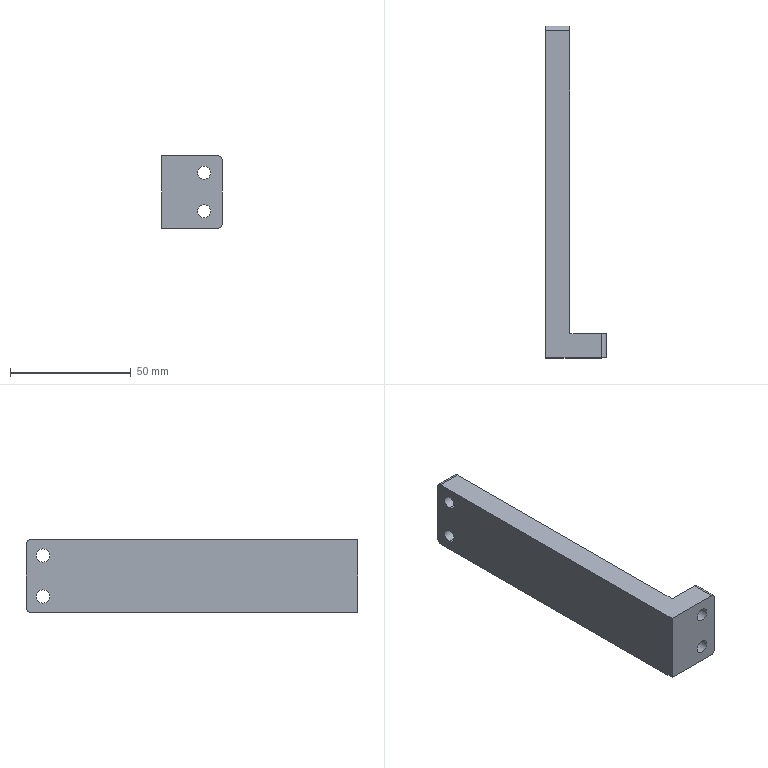Component | SolidWorks | ZHDJ-G002-1 | 1 solid | 32 faces | box 25 x 137.5 x 30 mm | volume 43516 mm3 | cylinder 20 | plane 12 | commonest cylinder face diameters 10 x8 5.5 x8 4 x4
build123d program:
from build123d import *

# Parameters (mm, degrees)
EXTRUDE_THIN1_DEPTH = 15
FILLET1_R           = 2


with BuildPart() as part:
    # Sketch1 → Extrude-Thin1 (new, symmetric)
    with BuildSketch(Plane(origin=(0, 0, 0), x_dir=(0, 0, -1), z_dir=(1, 0, 0))):
        Polygon((15, 0), (0, 0), (0, 127.5), (-10, 127.5), (-10, -10), (15, -10), align=None)
    extrude(amount=EXTRUDE_THIN1_DEPTH, both=True)

    # Fillet1
    fillet1_edges = [part.edges().sort_by_distance(p)[0] for p in [
        (15, 127.5, 5),
        (-15, 127.5, 5),
        (-15, -5, -15),
        (15, -5, -15),
    ]]
    fillet(fillet1_edges, radius=FILLET1_R)

    # Sketch3 → Hole Size _According to_ Type 1 of Hexag (revolve, cut)
    with BuildSketch(Plane(origin=(-8, 0, -7.5), x_dir=(0, 0, 1), z_dir=(1, 0, 0))):
        Polygon((0, 0), (0, 15.652), (2.75, 14), (2.75, 5.7), (5, 5.7), (5, 0), align=None)
    hole_size_according_to_type_1_of_hexag = revolve(axis=Axis((-8, 6.35, -7.5), (0, -1, 0)), mode=Mode.SUBTRACT)

    # Mirror1: Hole Size _According to_ Type 1 of Hexag across plane
    add(hole_size_according_to_type_1_of_hexag.mirror(Plane(origin=(0, 0, 0), x_dir=(0, 0, 1), z_dir=(1, 0, 0))), mode=Mode.SUBTRACT)

    # Sketch5 → Hole Size_ according to_ Type 2 Hex Sock (revolve, cut)
    with BuildSketch(Plane(origin=(8.5, 120.498, 0), x_dir=(0, 1, 0), z_dir=(1, 0, 0))):
        Polygon((0, 0), (0, 15.652), (2.75, 14), (2.75, 5.7), (5, 5.7), (5, 0), align=None)
    hole_size_according_to_type_2_hex_sock = revolve(axis=Axis((8.5, 120.498, -6.35), (0, 0, 1)), mode=Mode.SUBTRACT)

    # Mirror2: Hole Size_ according to_ Type 2 Hex Sock across plane
    add(hole_size_according_to_type_2_hex_sock.mirror(Plane(origin=(0, 0, 0), x_dir=(0, 0, 1), z_dir=(1, 0, 0))), mode=Mode.SUBTRACT)


solid = part.part

# Placed as in the assembly
solid = solid.moved(Location((56, -137.498, -110), (0, -90, 0)))
STEP:
#1=COLOUR_RGB('',0.7922,0.8196,0.9333);
#2=FILL_AREA_STYLE_COLOUR('',#1);
#3=FILL_AREA_STYLE('',(#2));
#4=SURFACE_STYLE_FILL_AREA(#3);
#5=SURFACE_SIDE_STYLE('',(#4));
#6=SURFACE_STYLE_USAGE(.BOTH.,#5);
#7=PRESENTATION_STYLE_ASSIGNMENT((#6));
#8=CARTESIAN_POINT('',(1.98,-0.6693,-4.469));
#9=VERTEX_POINT('',#8);
#10=CARTESIAN_POINT('',(1.98,-0.6693,-4.862));
#11=VERTEX_POINT('',#10);
#12=CARTESIAN_POINT('',(1.98,-0.6693,-4.665));
#13=DIRECTION('',(1.,0.,0.));
#14=DIRECTION('',(0.,0.,-1.));
#15=AXIS2_PLACEMENT_3D('',#12,#13,#14);
#16=CIRCLE('',#15,0.1969);
#17=EDGE_CURVE('',#9,#11,#16,.T.);
#18=ORIENTED_EDGE('',*,*,#17,.F.);
#19=CARTESIAN_POINT('',(2.205,-0.6693,-4.469));
#20=VERTEX_POINT('',#19);
#21=CARTESIAN_POINT('',(2.205,-0.6693,-4.469));
#22=DIRECTION('',(1.,0.,0.));
#23=VECTOR('',#22,39.37);
#24=LINE('',#21,#23);
#25=EDGE_CURVE('',#9,#20,#24,.T.);
#26=ORIENTED_EDGE('',*,*,#25,.T.);
#27=CARTESIAN_POINT('',(2.205,-0.6693,-4.862));
#28=VERTEX_POINT('',#27);
#29=CARTESIAN_POINT('',(2.205,-0.6693,-4.665));
#30=DIRECTION('',(1.,0.,0.));
#31=DIRECTION('',(0.,0.,-1.));
#32=AXIS2_PLACEMENT_3D('',#29,#30,#31);
#33=CIRCLE('',#32,0.1969);
#34=EDGE_CURVE('',#20,#28,#33,.T.);
#35=ORIENTED_EDGE('',*,*,#34,.T.);
#36=CARTESIAN_POINT('',(2.205,-0.6693,-4.862));
#37=DIRECTION('',(1.,0.,0.));
#38=VECTOR('',#37,39.37);
#39=LINE('',#36,#38);
#40=EDGE_CURVE('',#11,#28,#39,.T.);
#41=ORIENTED_EDGE('',*,*,#40,.F.);
#42=EDGE_LOOP('',(#18,#26,#35,#41));
#43=FACE_OUTER_BOUND('',#42,.T.);
#44=CARTESIAN_POINT('',(2.205,-0.6693,-4.665));
#45=DIRECTION('',(1.,0.,0.));
#46=DIRECTION('',(0.,0.,-1.));
#47=AXIS2_PLACEMENT_3D('',#44,#45,#46);
#48=CYLINDRICAL_SURFACE('',#47,0.1969);
#49=ADVANCED_FACE('',(#43),#48,.F.);
#50=CARTESIAN_POINT('',(1.811,-0.6693,-4.557));
#51=VERTEX_POINT('',#50);
#52=CARTESIAN_POINT('',(1.811,-0.6693,-4.774));
#53=VERTEX_POINT('',#52);
#54=CARTESIAN_POINT('',(1.811,-0.6693,-4.665));
#55=DIRECTION('',(1.,0.,0.));
#56=DIRECTION('',(0.,0.,-1.));
#57=AXIS2_PLACEMENT_3D('',#54,#55,#56);
#58=CIRCLE('',#57,0.1083);
#59=EDGE_CURVE('',#51,#53,#58,.T.);
#60=ORIENTED_EDGE('',*,*,#59,.F.);
#61=CARTESIAN_POINT('',(1.98,-0.6693,-4.557));
#62=VERTEX_POINT('',#61);
#63=CARTESIAN_POINT('',(2.205,-0.6693,-4.557));
#64=DIRECTION('',(1.,0.,0.));
#65=VECTOR('',#64,39.37);
#66=LINE('',#63,#65);
#67=EDGE_CURVE('',#51,#62,#66,.T.);
#68=ORIENTED_EDGE('',*,*,#67,.T.);
#69=CARTESIAN_POINT('',(1.98,-0.6693,-4.774));
#70=VERTEX_POINT('',#69);
#71=CARTESIAN_POINT('',(1.98,-0.6693,-4.665));
#72=DIRECTION('',(1.,0.,0.));
#73=DIRECTION('',(0.,0.,-1.));
#74=AXIS2_PLACEMENT_3D('',#71,#72,#73);
#75=CIRCLE('',#74,0.1083);
#76=EDGE_CURVE('',#62,#70,#75,.T.);
#77=ORIENTED_EDGE('',*,*,#76,.T.);
#78=CARTESIAN_POINT('',(2.205,-0.6693,-4.774));
#79=DIRECTION('',(1.,0.,0.));
#80=VECTOR('',#79,39.37);
#81=LINE('',#78,#80);
#82=EDGE_CURVE('',#53,#70,#81,.T.);
#83=ORIENTED_EDGE('',*,*,#82,.F.);
#84=EDGE_LOOP('',(#60,#68,#77,#83));
#85=FACE_OUTER_BOUND('',#84,.T.);
#86=CARTESIAN_POINT('',(2.205,-0.6693,-4.665));
#87=DIRECTION('',(1.,0.,0.));
#88=DIRECTION('',(0.,0.,-1.));
#89=AXIS2_PLACEMENT_3D('',#86,#87,#88);
#90=CYLINDRICAL_SURFACE('',#89,0.1083);
#91=ADVANCED_FACE('',(#85),#90,.F.);
#92=CARTESIAN_POINT('',(1.98,-0.6693,-3.799));
#93=VERTEX_POINT('',#92);
#94=CARTESIAN_POINT('',(1.98,-0.6693,-4.193));
#95=VERTEX_POINT('',#94);
#96=CARTESIAN_POINT('',(1.98,-0.6693,-3.996));
#97=DIRECTION('',(1.,0.,0.));
#98=DIRECTION('',(0.,0.,-1.));
#99=AXIS2_PLACEMENT_3D('',#96,#97,#98);
#100=CIRCLE('',#99,0.1969);
#101=EDGE_CURVE('',#93,#95,#100,.T.);
#102=ORIENTED_EDGE('',*,*,#101,.F.);
#103=CARTESIAN_POINT('',(2.205,-0.6693,-3.799));
#104=VERTEX_POINT('',#103);
#105=CARTESIAN_POINT('',(2.205,-0.6693,-3.799));
#106=DIRECTION('',(1.,0.,0.));
#107=VECTOR('',#106,39.37);
#108=LINE('',#105,#107);
#109=EDGE_CURVE('',#93,#104,#108,.T.);
#110=ORIENTED_EDGE('',*,*,#109,.T.);
#111=CARTESIAN_POINT('',(2.205,-0.6693,-4.193));
#112=VERTEX_POINT('',#111);
#113=CARTESIAN_POINT('',(2.205,-0.6693,-3.996));
#114=DIRECTION('',(1.,0.,0.));
#115=DIRECTION('',(0.,0.,-1.));
#116=AXIS2_PLACEMENT_3D('',#113,#114,#115);
#117=CIRCLE('',#116,0.1969);
#118=EDGE_CURVE('',#104,#112,#117,.T.);
#119=ORIENTED_EDGE('',*,*,#118,.T.);
#120=CARTESIAN_POINT('',(2.205,-0.6693,-4.193));
#121=DIRECTION('',(1.,0.,0.));
#122=VECTOR('',#121,39.37);
#123=LINE('',#120,#122);
#124=EDGE_CURVE('',#95,#112,#123,.T.);
#125=ORIENTED_EDGE('',*,*,#124,.F.);
#126=EDGE_LOOP('',(#102,#110,#119,#125));
#127=FACE_OUTER_BOUND('',#126,.T.);
#128=CARTESIAN_POINT('',(2.205,-0.6693,-3.996));
#129=DIRECTION('',(1.,0.,0.));
#130=DIRECTION('',(0.,0.,-1.));
#131=AXIS2_PLACEMENT_3D('',#128,#129,#130);
#132=CYLINDRICAL_SURFACE('',#131,0.1969);
#133=ADVANCED_FACE('',(#127),#132,.F.);
#134=CARTESIAN_POINT('',(1.811,-0.6693,-3.888));
#135=VERTEX_POINT('',#134);
#136=CARTESIAN_POINT('',(1.811,-0.6693,-4.104));
#137=VERTEX_POINT('',#136);
#138=CARTESIAN_POINT('',(1.811,-0.6693,-3.996));
#139=DIRECTION('',(1.,0.,0.));
#140=DIRECTION('',(0.,0.,-1.));
#141=AXIS2_PLACEMENT_3D('',#138,#139,#140);
#142=CIRCLE('',#141,0.1083);
#143=EDGE_CURVE('',#135,#137,#142,.T.);
#144=ORIENTED_EDGE('',*,*,#143,.F.);
#145=CARTESIAN_POINT('',(1.98,-0.6693,-3.888));
#146=VERTEX_POINT('',#145);
#147=CARTESIAN_POINT('',(2.205,-0.6693,-3.888));
#148=DIRECTION('',(1.,0.,0.));
#149=VECTOR('',#148,39.37);
#150=LINE('',#147,#149);
#151=EDGE_CURVE('',#135,#146,#150,.T.);
#152=ORIENTED_EDGE('',*,*,#151,.T.);
#153=CARTESIAN_POINT('',(1.98,-0.6693,-4.104));
#154=VERTEX_POINT('',#153);
#155=CARTESIAN_POINT('',(1.98,-0.6693,-3.996));
#156=DIRECTION('',(1.,0.,0.));
#157=DIRECTION('',(0.,0.,-1.));
#158=AXIS2_PLACEMENT_3D('',#155,#156,#157);
#159=CIRCLE('',#158,0.1083);
#160=EDGE_CURVE('',#146,#154,#159,.T.);
#161=ORIENTED_EDGE('',*,*,#160,.T.);
#162=CARTESIAN_POINT('',(2.205,-0.6693,-4.104));
#163=DIRECTION('',(1.,0.,0.));
#164=VECTOR('',#163,39.37);
#165=LINE('',#162,#164);
#166=EDGE_CURVE('',#137,#154,#165,.T.);
#167=ORIENTED_EDGE('',*,*,#166,.F.);
#168=EDGE_LOOP('',(#144,#152,#161,#167));
#169=FACE_OUTER_BOUND('',#168,.T.);
#170=CARTESIAN_POINT('',(2.205,-0.6693,-3.996));
#171=DIRECTION('',(1.,0.,0.));
#172=DIRECTION('',(0.,0.,-1.));
#173=AXIS2_PLACEMENT_3D('',#170,#171,#172);
#174=CYLINDRICAL_SURFACE('',#173,0.1083);
#175=ADVANCED_FACE('',(#169),#174,.F.);
#176=CARTESIAN_POINT('',(2.697,-5.638,-4.016));
#177=VERTEX_POINT('',#176);
#178=CARTESIAN_POINT('',(2.303,-5.638,-4.016));
#179=VERTEX_POINT('',#178);
#180=CARTESIAN_POINT('',(2.5,-5.638,-4.016));
#181=DIRECTION('',(0.,1.,0.));
#182=DIRECTION('',(-1.,0.,0.));
#183=AXIS2_PLACEMENT_3D('',#180,#181,#182);
#184=CIRCLE('',#183,0.1969);
#185=EDGE_CURVE('',#177,#179,#184,.T.);
#186=ORIENTED_EDGE('',*,*,#185,.F.);
#187=CARTESIAN_POINT('',(2.697,-5.413,-4.016));
#188=VERTEX_POINT('',#187);
#189=CARTESIAN_POINT('',(2.697,-5.413,-4.016));
#190=DIRECTION('',(0.,1.,0.));
#191=VECTOR('',#190,39.37);
#192=LINE('',#189,#191);
#193=EDGE_CURVE('',#177,#188,#192,.T.);
#194=ORIENTED_EDGE('',*,*,#193,.T.);
#195=CARTESIAN_POINT('',(2.303,-5.413,-4.016));
#196=VERTEX_POINT('',#195);
#197=CARTESIAN_POINT('',(2.5,-5.413,-4.016));
#198=DIRECTION('',(0.,1.,0.));
#199=DIRECTION('',(-1.,0.,0.));
#200=AXIS2_PLACEMENT_3D('',#197,#198,#199);
#201=CIRCLE('',#200,0.1969);
#202=EDGE_CURVE('',#188,#196,#201,.T.);
#203=ORIENTED_EDGE('',*,*,#202,.T.);
#204=CARTESIAN_POINT('',(2.303,-5.413,-4.016));
#205=DIRECTION('',(0.,1.,0.));
#206=VECTOR('',#205,39.37);
#207=LINE('',#204,#206);
#208=EDGE_CURVE('',#179,#196,#207,.T.);
#209=ORIENTED_EDGE('',*,*,#208,.F.);
#210=EDGE_LOOP('',(#186,#194,#203,#209));
#211=FACE_OUTER_BOUND('',#210,.T.);
#212=CARTESIAN_POINT('',(2.5,-5.413,-4.016));
#213=DIRECTION('',(0.,1.,0.));
#214=DIRECTION('',(-1.,0.,0.));
#215=AXIS2_PLACEMENT_3D('',#212,#213,#214);
#216=CYLINDRICAL_SURFACE('',#215,0.1969);
#217=ADVANCED_FACE('',(#211),#216,.F.);
#218=CARTESIAN_POINT('',(2.608,-5.807,-4.016));
#219=VERTEX_POINT('',#218);
#220=CARTESIAN_POINT('',(2.392,-5.807,-4.016));
#221=VERTEX_POINT('',#220);
#222=CARTESIAN_POINT('',(2.5,-5.807,-4.016));
#223=DIRECTION('',(0.,1.,0.));
#224=DIRECTION('',(-1.,0.,0.));
#225=AXIS2_PLACEMENT_3D('',#222,#223,#224);
#226=CIRCLE('',#225,0.1083);
#227=EDGE_CURVE('',#219,#221,#226,.T.);
#228=ORIENTED_EDGE('',*,*,#227,.F.);
#229=CARTESIAN_POINT('',(2.608,-5.638,-4.016));
#230=VERTEX_POINT('',#229);
#231=CARTESIAN_POINT('',(2.608,-5.413,-4.016));
#232=DIRECTION('',(0.,1.,0.));
#233=VECTOR('',#232,39.37);
#234=LINE('',#231,#233);
#235=EDGE_CURVE('',#219,#230,#234,.T.);
#236=ORIENTED_EDGE('',*,*,#235,.T.);
#237=CARTESIAN_POINT('',(2.392,-5.638,-4.016));
#238=VERTEX_POINT('',#237);
#239=CARTESIAN_POINT('',(2.5,-5.638,-4.016));
#240=DIRECTION('',(0.,1.,0.));
#241=DIRECTION('',(-1.,0.,0.));
#242=AXIS2_PLACEMENT_3D('',#239,#240,#241);
#243=CIRCLE('',#242,0.1083);
#244=EDGE_CURVE('',#230,#238,#243,.T.);
#245=ORIENTED_EDGE('',*,*,#244,.T.);
#246=CARTESIAN_POINT('',(2.392,-5.413,-4.016));
#247=DIRECTION('',(0.,1.,0.));
#248=VECTOR('',#247,39.37);
#249=LINE('',#246,#248);
#250=EDGE_CURVE('',#221,#238,#249,.T.);
#251=ORIENTED_EDGE('',*,*,#250,.F.);
#252=EDGE_LOOP('',(#228,#236,#245,#251));
#253=FACE_OUTER_BOUND('',#252,.T.);
#254=CARTESIAN_POINT('',(2.5,-5.413,-4.016));
#255=DIRECTION('',(0.,1.,0.));
#256=DIRECTION('',(-1.,0.,0.));
#257=AXIS2_PLACEMENT_3D('',#254,#255,#256);
#258=CYLINDRICAL_SURFACE('',#257,0.1083);
#259=ADVANCED_FACE('',(#253),#258,.F.);
#260=CARTESIAN_POINT('',(2.697,-5.638,-4.646));
#261=VERTEX_POINT('',#260);
#262=CARTESIAN_POINT('',(2.303,-5.638,-4.646));
#263=VERTEX_POINT('',#262);
#264=CARTESIAN_POINT('',(2.5,-5.638,-4.646));
#265=DIRECTION('',(0.,1.,0.));
#266=DIRECTION('',(-1.,0.,0.));
#267=AXIS2_PLACEMENT_3D('',#264,#265,#266);
#268=CIRCLE('',#267,0.1969);
#269=EDGE_CURVE('',#261,#263,#268,.T.);
#270=ORIENTED_EDGE('',*,*,#269,.F.);
#271=CARTESIAN_POINT('',(2.697,-5.413,-4.646));
#272=VERTEX_POINT('',#271);
#273=CARTESIAN_POINT('',(2.697,-5.413,-4.646));
#274=DIRECTION('',(0.,1.,0.));
#275=VECTOR('',#274,39.37);
#276=LINE('',#273,#275);
#277=EDGE_CURVE('',#261,#272,#276,.T.);
#278=ORIENTED_EDGE('',*,*,#277,.T.);
#279=CARTESIAN_POINT('',(2.303,-5.413,-4.646));
#280=VERTEX_POINT('',#279);
#281=CARTESIAN_POINT('',(2.5,-5.413,-4.646));
#282=DIRECTION('',(0.,1.,0.));
#283=DIRECTION('',(-1.,0.,0.));
#284=AXIS2_PLACEMENT_3D('',#281,#282,#283);
#285=CIRCLE('',#284,0.1969);
#286=EDGE_CURVE('',#272,#280,#285,.T.);
#287=ORIENTED_EDGE('',*,*,#286,.T.);
#288=CARTESIAN_POINT('',(2.303,-5.413,-4.646));
#289=DIRECTION('',(0.,1.,0.));
#290=VECTOR('',#289,39.37);
#291=LINE('',#288,#290);
#292=EDGE_CURVE('',#263,#280,#291,.T.);
#293=ORIENTED_EDGE('',*,*,#292,.F.);
#294=EDGE_LOOP('',(#270,#278,#287,#293));
#295=FACE_OUTER_BOUND('',#294,.T.);
#296=CARTESIAN_POINT('',(2.5,-5.413,-4.646));
#297=DIRECTION('',(0.,1.,0.));
#298=DIRECTION('',(-1.,0.,0.));
#299=AXIS2_PLACEMENT_3D('',#296,#297,#298);
#300=CYLINDRICAL_SURFACE('',#299,0.1969);
#301=ADVANCED_FACE('',(#295),#300,.F.);
#302=CARTESIAN_POINT('',(2.608,-5.807,-4.646));
#303=VERTEX_POINT('',#302);
#304=CARTESIAN_POINT('',(2.392,-5.807,-4.646));
#305=VERTEX_POINT('',#304);
#306=CARTESIAN_POINT('',(2.5,-5.807,-4.646));
#307=DIRECTION('',(0.,1.,0.));
#308=DIRECTION('',(-1.,0.,0.));
#309=AXIS2_PLACEMENT_3D('',#306,#307,#308);
#310=CIRCLE('',#309,0.1083);
#311=EDGE_CURVE('',#303,#305,#310,.T.);
#312=ORIENTED_EDGE('',*,*,#311,.F.);
#313=CARTESIAN_POINT('',(2.608,-5.638,-4.646));
#314=VERTEX_POINT('',#313);
#315=CARTESIAN_POINT('',(2.608,-5.413,-4.646));
#316=DIRECTION('',(0.,1.,0.));
#317=VECTOR('',#316,39.37);
#318=LINE('',#315,#317);
#319=EDGE_CURVE('',#303,#314,#318,.T.);
#320=ORIENTED_EDGE('',*,*,#319,.T.);
#321=CARTESIAN_POINT('',(2.392,-5.638,-4.646));
#322=VERTEX_POINT('',#321);
#323=CARTESIAN_POINT('',(2.5,-5.638,-4.646));
#324=DIRECTION('',(0.,1.,0.));
#325=DIRECTION('',(-1.,0.,0.));
#326=AXIS2_PLACEMENT_3D('',#323,#324,#325);
#327=CIRCLE('',#326,0.1083);
#328=EDGE_CURVE('',#314,#322,#327,.T.);
#329=ORIENTED_EDGE('',*,*,#328,.T.);
#330=CARTESIAN_POINT('',(2.392,-5.413,-4.646));
#331=DIRECTION('',(0.,1.,0.));
#332=VECTOR('',#331,39.37);
#333=LINE('',#330,#332);
#334=EDGE_CURVE('',#305,#322,#333,.T.);
#335=ORIENTED_EDGE('',*,*,#334,.F.);
#336=EDGE_LOOP('',(#312,#320,#329,#335));
#337=FACE_OUTER_BOUND('',#336,.T.);
#338=CARTESIAN_POINT('',(2.5,-5.413,-4.646));
#339=DIRECTION('',(0.,1.,0.));
#340=DIRECTION('',(-1.,0.,0.));
#341=AXIS2_PLACEMENT_3D('',#338,#339,#340);
#342=CYLINDRICAL_SURFACE('',#341,0.1083);
#343=ADVANCED_FACE('',(#337),#342,.F.);
#344=CARTESIAN_POINT('',(2.5,-5.807,-4.016));
#345=DIRECTION('',(0.,1.,0.));
#346=DIRECTION('',(-1.,0.,0.));
#347=AXIS2_PLACEMENT_3D('',#344,#345,#346);
#348=CIRCLE('',#347,0.1083);
#349=EDGE_CURVE('',#221,#219,#348,.T.);
#350=ORIENTED_EDGE('',*,*,#349,.T.);
#351=ORIENTED_EDGE('',*,*,#227,.T.);
#352=EDGE_LOOP('',(#350,#351));
#353=FACE_BOUND('',#352,.T.);
#354=CARTESIAN_POINT('',(2.5,-5.807,-4.646));
#355=DIRECTION('',(0.,1.,0.));
#356=DIRECTION('',(-1.,0.,0.));
#357=AXIS2_PLACEMENT_3D('',#354,#355,#356);
#358=CIRCLE('',#357,0.1083);
#359=EDGE_CURVE('',#305,#303,#358,.T.);
#360=ORIENTED_EDGE('',*,*,#359,.T.);
#361=ORIENTED_EDGE('',*,*,#311,.T.);
#362=EDGE_LOOP('',(#360,#361));
#363=FACE_BOUND('',#362,.T.);
#364=CARTESIAN_POINT('',(2.795,-5.807,-3.819));
#365=VERTEX_POINT('',#364);
#366=CARTESIAN_POINT('',(2.795,-5.807,-4.843));
#367=VERTEX_POINT('',#366);
#368=CARTESIAN_POINT('',(2.795,-5.807,-3.74));
#369=DIRECTION('',(0.,0.,-1.));
#370=VECTOR('',#369,39.37);
#371=LINE('',#368,#370);
#372=EDGE_CURVE('',#365,#367,#371,.T.);
#373=ORIENTED_EDGE('',*,*,#372,.F.);
#374=CARTESIAN_POINT('',(2.717,-5.807,-3.74));
#375=VERTEX_POINT('',#374);
#376=CARTESIAN_POINT('',(2.717,-5.807,-3.819));
#377=DIRECTION('',(0.,-1.,0.));
#378=DIRECTION('',(-1.,0.,0.));
#379=AXIS2_PLACEMENT_3D('',#376,#377,#378);
#380=CIRCLE('',#379,0.07874);
#381=EDGE_CURVE('',#365,#375,#380,.T.);
#382=ORIENTED_EDGE('',*,*,#381,.T.);
#383=CARTESIAN_POINT('',(1.811,-5.807,-3.74));
#384=VERTEX_POINT('',#383);
#385=CARTESIAN_POINT('',(2.205,-5.807,-3.74));
#386=DIRECTION('',(1.,0.,0.));
#387=VECTOR('',#386,39.37);
#388=LINE('',#385,#387);
#389=EDGE_CURVE('',#384,#375,#388,.T.);
#390=ORIENTED_EDGE('',*,*,#389,.F.);
#391=CARTESIAN_POINT('',(1.811,-5.807,-4.921));
#392=VERTEX_POINT('',#391);
#393=CARTESIAN_POINT('',(1.811,-5.807,-3.74));
#394=DIRECTION('',(0.,0.,-1.));
#395=VECTOR('',#394,39.37);
#396=LINE('',#393,#395);
#397=EDGE_CURVE('',#384,#392,#396,.T.);
#398=ORIENTED_EDGE('',*,*,#397,.T.);
#399=CARTESIAN_POINT('',(2.717,-5.807,-4.921));
#400=VERTEX_POINT('',#399);
#401=CARTESIAN_POINT('',(2.205,-5.807,-4.921));
#402=DIRECTION('',(1.,0.,0.));
#403=VECTOR('',#402,39.37);
#404=LINE('',#401,#403);
#405=EDGE_CURVE('',#392,#400,#404,.T.);
#406=ORIENTED_EDGE('',*,*,#405,.T.);
#407=CARTESIAN_POINT('',(2.717,-5.807,-4.843));
#408=DIRECTION('',(0.,-1.,0.));
#409=DIRECTION('',(-1.,0.,0.));
#410=AXIS2_PLACEMENT_3D('',#407,#408,#409);
#411=CIRCLE('',#410,0.07874);
#412=EDGE_CURVE('',#400,#367,#411,.T.);
#413=ORIENTED_EDGE('',*,*,#412,.T.);
#414=EDGE_LOOP('',(#373,#382,#390,#398,#406,#413));
#415=FACE_OUTER_BOUND('',#414,.T.);
#416=CARTESIAN_POINT('',(2.205,-5.807,-3.74));
#417=DIRECTION('',(0.,1.,0.));
#418=DIRECTION('',(-1.,0.,0.));
#419=AXIS2_PLACEMENT_3D('',#416,#417,#418);
#420=PLANE('',#419);
#421=ADVANCED_FACE('',(#353,#363,#415),#420,.F.);
#422=CARTESIAN_POINT('',(2.795,-5.413,-3.819));
#423=VERTEX_POINT('',#422);
#424=CARTESIAN_POINT('',(2.795,-5.413,-4.843));
#425=VERTEX_POINT('',#424);
#426=CARTESIAN_POINT('',(2.795,-5.413,-3.74));
#427=DIRECTION('',(0.,0.,-1.));
#428=VECTOR('',#427,39.37);
#429=LINE('',#426,#428);
#430=EDGE_CURVE('',#423,#425,#429,.T.);
#431=ORIENTED_EDGE('',*,*,#430,.F.);
#432=CARTESIAN_POINT('',(2.795,-5.807,-3.819));
#433=DIRECTION('',(0.,-1.,0.));
#434=VECTOR('',#433,39.37);
#435=LINE('',#432,#434);
#436=EDGE_CURVE('',#423,#365,#435,.T.);
#437=ORIENTED_EDGE('',*,*,#436,.T.);
#438=ORIENTED_EDGE('',*,*,#372,.T.);
#439=CARTESIAN_POINT('',(2.795,-5.413,-4.843));
#440=DIRECTION('',(0.,1.,0.));
#441=VECTOR('',#440,39.37);
#442=LINE('',#439,#441);
#443=EDGE_CURVE('',#367,#425,#442,.T.);
#444=ORIENTED_EDGE('',*,*,#443,.T.);
#445=EDGE_LOOP('',(#431,#437,#438,#444));
#446=FACE_OUTER_BOUND('',#445,.T.);
#447=CARTESIAN_POINT('',(2.795,-5.413,-3.74));
#448=DIRECTION('',(1.,0.,0.));
#449=DIRECTION('',(0.,0.,-1.));
#450=AXIS2_PLACEMENT_3D('',#447,#448,#449);
#451=PLANE('',#450);
#452=ADVANCED_FACE('',(#446),#451,.T.);
#453=CARTESIAN_POINT('',(2.5,-5.413,-4.016));
#454=DIRECTION('',(0.,1.,0.));
#455=DIRECTION('',(-1.,0.,0.));
#456=AXIS2_PLACEMENT_3D('',#453,#454,#455);
#457=CIRCLE('',#456,0.1969);
#458=EDGE_CURVE('',#196,#188,#457,.T.);
#459=ORIENTED_EDGE('',*,*,#458,.F.);
#460=ORIENTED_EDGE('',*,*,#202,.F.);
#461=EDGE_LOOP('',(#459,#460));
#462=FACE_BOUND('',#461,.T.);
#463=CARTESIAN_POINT('',(2.5,-5.413,-4.646));
#464=DIRECTION('',(0.,1.,0.));
#465=DIRECTION('',(-1.,0.,0.));
#466=AXIS2_PLACEMENT_3D('',#463,#464,#465);
#467=CIRCLE('',#466,0.1969);
#468=EDGE_CURVE('',#280,#272,#467,.T.);
#469=ORIENTED_EDGE('',*,*,#468,.F.);
#470=ORIENTED_EDGE('',*,*,#286,.F.);
#471=EDGE_LOOP('',(#469,#470));
#472=FACE_BOUND('',#471,.T.);
#473=CARTESIAN_POINT('',(2.205,-5.413,-3.74));
#474=VERTEX_POINT('',#473);
#475=CARTESIAN_POINT('',(2.717,-5.413,-3.74));
#476=VERTEX_POINT('',#475);
#477=CARTESIAN_POINT('',(2.205,-5.413,-3.74));
#478=DIRECTION('',(1.,0.,0.));
#479=VECTOR('',#478,39.37);
#480=LINE('',#477,#479);
#481=EDGE_CURVE('',#474,#476,#480,.T.);
#482=ORIENTED_EDGE('',*,*,#481,.T.);
#483=CARTESIAN_POINT('',(2.717,-5.413,-3.819));
#484=DIRECTION('',(0.,1.,0.));
#485=DIRECTION('',(-1.,0.,0.));
#486=AXIS2_PLACEMENT_3D('',#483,#484,#485);
#487=CIRCLE('',#486,0.07874);
#488=EDGE_CURVE('',#476,#423,#487,.T.);
#489=ORIENTED_EDGE('',*,*,#488,.T.);
#490=ORIENTED_EDGE('',*,*,#430,.T.);
#491=CARTESIAN_POINT('',(2.717,-5.413,-4.921));
#492=VERTEX_POINT('',#491);
#493=CARTESIAN_POINT('',(2.717,-5.413,-4.843));
#494=DIRECTION('',(0.,1.,0.));
#495=DIRECTION('',(-1.,0.,0.));
#496=AXIS2_PLACEMENT_3D('',#493,#494,#495);
#497=CIRCLE('',#496,0.07874);
#498=EDGE_CURVE('',#425,#492,#497,.T.);
#499=ORIENTED_EDGE('',*,*,#498,.T.);
#500=CARTESIAN_POINT('',(2.205,-5.413,-4.921));
#501=VERTEX_POINT('',#500);
#502=CARTESIAN_POINT('',(2.205,-5.413,-4.921));
#503=DIRECTION('',(1.,0.,0.));
#504=VECTOR('',#503,39.37);
#505=LINE('',#502,#504);
#506=EDGE_CURVE('',#501,#492,#505,.T.);
#507=ORIENTED_EDGE('',*,*,#506,.F.);
#508=CARTESIAN_POINT('',(2.205,-5.413,-3.74));
#509=DIRECTION('',(0.,0.,-1.));
#510=VECTOR('',#509,39.37);
#511=LINE('',#508,#510);
#512=EDGE_CURVE('',#474,#501,#511,.T.);
#513=ORIENTED_EDGE('',*,*,#512,.F.);
#514=EDGE_LOOP('',(#482,#489,#490,#499,#507,#513));
#515=FACE_OUTER_BOUND('',#514,.T.);
#516=CARTESIAN_POINT('',(2.205,-5.413,-3.74));
#517=DIRECTION('',(0.,1.,0.));
#518=DIRECTION('',(-1.,0.,0.));
#519=AXIS2_PLACEMENT_3D('',#516,#517,#518);
#520=PLANE('',#519);
#521=ADVANCED_FACE('',(#462,#472,#515),#520,.T.);
#522=CARTESIAN_POINT('',(2.205,-0.6693,-4.665));
#523=DIRECTION('',(1.,0.,0.));
#524=DIRECTION('',(0.,0.,-1.));
#525=AXIS2_PLACEMENT_3D('',#522,#523,#524);
#526=CIRCLE('',#525,0.1969);
#527=EDGE_CURVE('',#28,#20,#526,.T.);
#528=ORIENTED_EDGE('',*,*,#527,.F.);
#529=ORIENTED_EDGE('',*,*,#34,.F.);
#530=EDGE_LOOP('',(#528,#529));
#531=FACE_BOUND('',#530,.T.);
#532=CARTESIAN_POINT('',(2.205,-0.6693,-3.996));
#533=DIRECTION('',(1.,0.,0.));
#534=DIRECTION('',(0.,0.,-1.));
#535=AXIS2_PLACEMENT_3D('',#532,#533,#534);
#536=CIRCLE('',#535,0.1969);
#537=EDGE_CURVE('',#112,#104,#536,.T.);
#538=ORIENTED_EDGE('',*,*,#537,.F.);
#539=ORIENTED_EDGE('',*,*,#118,.F.);
#540=EDGE_LOOP('',(#538,#539));
#541=FACE_BOUND('',#540,.T.);
#542=CARTESIAN_POINT('',(2.205,-0.4724,-4.921));
#543=VERTEX_POINT('',#542);
#544=CARTESIAN_POINT('',(2.205,-5.413,-4.921));
#545=DIRECTION('',(0.,-1.,0.));
#546=VECTOR('',#545,39.37);
#547=LINE('',#544,#546);
#548=EDGE_CURVE('',#543,#501,#547,.T.);
#549=ORIENTED_EDGE('',*,*,#548,.F.);
#550=CARTESIAN_POINT('',(2.205,-0.3936,-4.843));
#551=VERTEX_POINT('',#550);
#552=CARTESIAN_POINT('',(2.205,-0.4724,-4.843));
#553=DIRECTION('',(1.,0.,0.));
#554=DIRECTION('',(0.,0.,-1.));
#555=AXIS2_PLACEMENT_3D('',#552,#553,#554);
#556=CIRCLE('',#555,0.07874);
#557=EDGE_CURVE('',#543,#551,#556,.T.);
#558=ORIENTED_EDGE('',*,*,#557,.T.);
#559=CARTESIAN_POINT('',(2.205,-0.3936,-3.819));
#560=VERTEX_POINT('',#559);
#561=CARTESIAN_POINT('',(2.205,-0.3936,-3.74));
#562=DIRECTION('',(0.,0.,-1.));
#563=VECTOR('',#562,39.37);
#564=LINE('',#561,#563);
#565=EDGE_CURVE('',#560,#551,#564,.T.);
#566=ORIENTED_EDGE('',*,*,#565,.F.);
#567=CARTESIAN_POINT('',(2.205,-0.4724,-3.74));
#568=VERTEX_POINT('',#567);
#569=CARTESIAN_POINT('',(2.205,-0.4724,-3.819));
#570=DIRECTION('',(1.,0.,0.));
#571=DIRECTION('',(0.,0.,-1.));
#572=AXIS2_PLACEMENT_3D('',#569,#570,#571);
#573=CIRCLE('',#572,0.07874);
#574=EDGE_CURVE('',#560,#568,#573,.T.);
#575=ORIENTED_EDGE('',*,*,#574,.T.);
#576=CARTESIAN_POINT('',(2.205,-5.413,-3.74));
#577=DIRECTION('',(0.,-1.,0.));
#578=VECTOR('',#577,39.37);
#579=LINE('',#576,#578);
#580=EDGE_CURVE('',#568,#474,#579,.T.);
#581=ORIENTED_EDGE('',*,*,#580,.T.);
#582=ORIENTED_EDGE('',*,*,#512,.T.);
#583=EDGE_LOOP('',(#549,#558,#566,#575,#581,#582));
#584=FACE_OUTER_BOUND('',#583,.T.);
#585=CARTESIAN_POINT('',(2.205,-5.413,-3.74));
#586=DIRECTION('',(1.,0.,0.));
#587=DIRECTION('',(0.,0.,-1.));
#588=AXIS2_PLACEMENT_3D('',#585,#586,#587);
#589=PLANE('',#588);
#590=ADVANCED_FACE('',(#531,#541,#584),#589,.T.);
#591=ORIENTED_EDGE('',*,*,#565,.T.);
#592=CARTESIAN_POINT('',(1.811,-0.3936,-4.843));
#593=VERTEX_POINT('',#592);
#594=CARTESIAN_POINT('',(1.811,-0.3936,-4.843));
#595=DIRECTION('',(-1.,0.,0.));
#596=VECTOR('',#595,39.37);
#597=LINE('',#594,#596);
#598=EDGE_CURVE('',#551,#593,#597,.T.);
#599=ORIENTED_EDGE('',*,*,#598,.T.);
#600=CARTESIAN_POINT('',(1.811,-0.3936,-3.819));
#601=VERTEX_POINT('',#600);
#602=CARTESIAN_POINT('',(1.811,-0.3936,-3.74));
#603=DIRECTION('',(0.,0.,-1.));
#604=VECTOR('',#603,39.37);
#605=LINE('',#602,#604);
#606=EDGE_CURVE('',#601,#593,#605,.T.);
#607=ORIENTED_EDGE('',*,*,#606,.F.);
#608=CARTESIAN_POINT('',(2.205,-0.3936,-3.819));
#609=DIRECTION('',(1.,0.,0.));
#610=VECTOR('',#609,39.37);
#611=LINE('',#608,#610);
#612=EDGE_CURVE('',#601,#560,#611,.T.);
#613=ORIENTED_EDGE('',*,*,#612,.T.);
#614=EDGE_LOOP('',(#591,#599,#607,#613));
#615=FACE_OUTER_BOUND('',#614,.T.);
#616=CARTESIAN_POINT('',(1.811,-0.3936,-3.74));
#617=DIRECTION('',(0.,1.,0.));
#618=DIRECTION('',(-1.,0.,0.));
#619=AXIS2_PLACEMENT_3D('',#616,#617,#618);
#620=PLANE('',#619);
#621=ADVANCED_FACE('',(#615),#620,.T.);
#622=CARTESIAN_POINT('',(1.811,-0.6693,-4.665));
#623=DIRECTION('',(1.,0.,0.));
#624=DIRECTION('',(0.,0.,-1.));
#625=AXIS2_PLACEMENT_3D('',#622,#623,#624);
#626=CIRCLE('',#625,0.1083);
#627=EDGE_CURVE('',#53,#51,#626,.T.);
#628=ORIENTED_EDGE('',*,*,#627,.T.);
#629=ORIENTED_EDGE('',*,*,#59,.T.);
#630=EDGE_LOOP('',(#628,#629));
#631=FACE_BOUND('',#630,.T.);
#632=CARTESIAN_POINT('',(1.811,-0.6693,-3.996));
#633=DIRECTION('',(1.,0.,0.));
#634=DIRECTION('',(0.,0.,-1.));
#635=AXIS2_PLACEMENT_3D('',#632,#633,#634);
#636=CIRCLE('',#635,0.1083);
#637=EDGE_CURVE('',#137,#135,#636,.T.);
#638=ORIENTED_EDGE('',*,*,#637,.T.);
#639=ORIENTED_EDGE('',*,*,#143,.T.);
#640=EDGE_LOOP('',(#638,#639));
#641=FACE_BOUND('',#640,.T.);
#642=ORIENTED_EDGE('',*,*,#606,.T.);
#643=CARTESIAN_POINT('',(1.811,-0.4724,-4.921));
#644=VERTEX_POINT('',#643);
#645=CARTESIAN_POINT('',(1.811,-0.4724,-4.843));
#646=DIRECTION('',(-1.,0.,0.));
#647=DIRECTION('',(0.,0.,-1.));
#648=AXIS2_PLACEMENT_3D('',#645,#646,#647);
#649=CIRCLE('',#648,0.07874);
#650=EDGE_CURVE('',#593,#644,#649,.T.);
#651=ORIENTED_EDGE('',*,*,#650,.T.);
#652=CARTESIAN_POINT('',(1.811,-5.413,-4.921));
#653=DIRECTION('',(0.,-1.,0.));
#654=VECTOR('',#653,39.37);
#655=LINE('',#652,#654);
#656=EDGE_CURVE('',#644,#392,#655,.T.);
#657=ORIENTED_EDGE('',*,*,#656,.T.);
#658=ORIENTED_EDGE('',*,*,#397,.F.);
#659=CARTESIAN_POINT('',(1.811,-0.4724,-3.74));
#660=VERTEX_POINT('',#659);
#661=CARTESIAN_POINT('',(1.811,-5.413,-3.74));
#662=DIRECTION('',(0.,-1.,0.));
#663=VECTOR('',#662,39.37);
#664=LINE('',#661,#663);
#665=EDGE_CURVE('',#660,#384,#664,.T.);
#666=ORIENTED_EDGE('',*,*,#665,.F.);
#667=CARTESIAN_POINT('',(1.811,-0.4724,-3.819));
#668=DIRECTION('',(-1.,0.,0.));
#669=DIRECTION('',(0.,0.,-1.));
#670=AXIS2_PLACEMENT_3D('',#667,#668,#669);
#671=CIRCLE('',#670,0.07874);
#672=EDGE_CURVE('',#660,#601,#671,.T.);
#673=ORIENTED_EDGE('',*,*,#672,.T.);
#674=EDGE_LOOP('',(#642,#651,#657,#658,#666,#673));
#675=FACE_OUTER_BOUND('',#674,.T.);
#676=CARTESIAN_POINT('',(1.811,-5.413,-3.74));
#677=DIRECTION('',(1.,0.,0.));
#678=DIRECTION('',(0.,0.,-1.));
#679=AXIS2_PLACEMENT_3D('',#676,#677,#678);
#680=PLANE('',#679);
#681=ADVANCED_FACE('',(#631,#641,#675),#680,.F.);
#682=ORIENTED_EDGE('',*,*,#389,.T.);
#683=CARTESIAN_POINT('',(2.717,-5.413,-3.74));
#684=DIRECTION('',(0.,1.,0.));
#685=VECTOR('',#684,39.37);
#686=LINE('',#683,#685);
#687=EDGE_CURVE('',#375,#476,#686,.T.);
#688=ORIENTED_EDGE('',*,*,#687,.T.);
#689=ORIENTED_EDGE('',*,*,#481,.F.);
#690=ORIENTED_EDGE('',*,*,#580,.F.);
#691=CARTESIAN_POINT('',(1.811,-0.4724,-3.74));
#692=DIRECTION('',(-1.,0.,0.));
#693=VECTOR('',#692,39.37);
#694=LINE('',#691,#693);
#695=EDGE_CURVE('',#568,#660,#694,.T.);
#696=ORIENTED_EDGE('',*,*,#695,.T.);
#697=ORIENTED_EDGE('',*,*,#665,.T.);
#698=EDGE_LOOP('',(#682,#688,#689,#690,#696,#697));
#699=FACE_OUTER_BOUND('',#698,.T.);
#700=CARTESIAN_POINT('',(2.205,-5.413,-3.74));
#701=DIRECTION('',(0.,0.,-1.));
#702=DIRECTION('',(-1.,0.,0.));
#703=AXIS2_PLACEMENT_3D('',#700,#701,#702);
#704=PLANE('',#703);
#705=ADVANCED_FACE('',(#699),#704,.F.);
#706=ORIENTED_EDGE('',*,*,#506,.T.);
#707=CARTESIAN_POINT('',(2.717,-5.413,-4.921));
#708=DIRECTION('',(0.,-1.,0.));
#709=VECTOR('',#708,39.37);
#710=LINE('',#707,#709);
#711=EDGE_CURVE('',#492,#400,#710,.T.);
#712=ORIENTED_EDGE('',*,*,#711,.T.);
#713=ORIENTED_EDGE('',*,*,#405,.F.);
#714=ORIENTED_EDGE('',*,*,#656,.F.);
#715=CARTESIAN_POINT('',(2.205,-0.4724,-4.921));
#716=DIRECTION('',(1.,0.,0.));
#717=VECTOR('',#716,39.37);
#718=LINE('',#715,#717);
#719=EDGE_CURVE('',#644,#543,#718,.T.);
#720=ORIENTED_EDGE('',*,*,#719,.T.);
#721=ORIENTED_EDGE('',*,*,#548,.T.);
#722=EDGE_LOOP('',(#706,#712,#713,#714,#720,#721));
#723=FACE_OUTER_BOUND('',#722,.T.);
#724=CARTESIAN_POINT('',(2.205,-5.413,-4.921));
#725=DIRECTION('',(0.,0.,-1.));
#726=DIRECTION('',(-1.,0.,0.));
#727=AXIS2_PLACEMENT_3D('',#724,#725,#726);
#728=PLANE('',#727);
#729=ADVANCED_FACE('',(#723),#728,.T.);
#730=ORIENTED_EDGE('',*,*,#488,.F.);
#731=ORIENTED_EDGE('',*,*,#687,.F.);
#732=ORIENTED_EDGE('',*,*,#381,.F.);
#733=ORIENTED_EDGE('',*,*,#436,.F.);
#734=EDGE_LOOP('',(#730,#731,#732,#733));
#735=FACE_OUTER_BOUND('',#734,.T.);
#736=CARTESIAN_POINT('',(2.717,-5.413,-3.819));
#737=DIRECTION('',(0.,1.,0.));
#738=DIRECTION('',(-1.,0.,0.));
#739=AXIS2_PLACEMENT_3D('',#736,#737,#738);
#740=CYLINDRICAL_SURFACE('',#739,0.07874);
#741=ADVANCED_FACE('',(#735),#740,.T.);
#742=ORIENTED_EDGE('',*,*,#498,.F.);
#743=ORIENTED_EDGE('',*,*,#443,.F.);
#744=ORIENTED_EDGE('',*,*,#412,.F.);
#745=ORIENTED_EDGE('',*,*,#711,.F.);
#746=EDGE_LOOP('',(#742,#743,#744,#745));
#747=FACE_OUTER_BOUND('',#746,.T.);
#748=CARTESIAN_POINT('',(2.717,-5.413,-4.843));
#749=DIRECTION('',(0.,-1.,0.));
#750=DIRECTION('',(1.,0.,0.));
#751=AXIS2_PLACEMENT_3D('',#748,#749,#750);
#752=CYLINDRICAL_SURFACE('',#751,0.07874);
#753=ADVANCED_FACE('',(#747),#752,.T.);
#754=ORIENTED_EDGE('',*,*,#650,.F.);
#755=ORIENTED_EDGE('',*,*,#598,.F.);
#756=ORIENTED_EDGE('',*,*,#557,.F.);
#757=ORIENTED_EDGE('',*,*,#719,.F.);
#758=EDGE_LOOP('',(#754,#755,#756,#757));
#759=FACE_OUTER_BOUND('',#758,.T.);
#760=CARTESIAN_POINT('',(2.205,-0.4724,-4.843));
#761=DIRECTION('',(1.,0.,0.));
#762=DIRECTION('',(0.,0.,-1.));
#763=AXIS2_PLACEMENT_3D('',#760,#761,#762);
#764=CYLINDRICAL_SURFACE('',#763,0.07874);
#765=ADVANCED_FACE('',(#759),#764,.T.);
#766=ORIENTED_EDGE('',*,*,#672,.F.);
#767=ORIENTED_EDGE('',*,*,#695,.F.);
#768=ORIENTED_EDGE('',*,*,#574,.F.);
#769=ORIENTED_EDGE('',*,*,#612,.F.);
#770=EDGE_LOOP('',(#766,#767,#768,#769));
#771=FACE_OUTER_BOUND('',#770,.T.);
#772=CARTESIAN_POINT('',(1.811,-0.4724,-3.819));
#773=DIRECTION('',(-1.,0.,0.));
#774=DIRECTION('',(0.,0.,1.));
#775=AXIS2_PLACEMENT_3D('',#772,#773,#774);
#776=CYLINDRICAL_SURFACE('',#775,0.07874);
#777=ADVANCED_FACE('',(#771),#776,.T.);
#778=ORIENTED_EDGE('',*,*,#319,.F.);
#779=ORIENTED_EDGE('',*,*,#359,.F.);
#780=ORIENTED_EDGE('',*,*,#334,.T.);
#781=CARTESIAN_POINT('',(2.5,-5.638,-4.646));
#782=DIRECTION('',(0.,1.,0.));
#783=DIRECTION('',(-1.,0.,0.));
#784=AXIS2_PLACEMENT_3D('',#781,#782,#783);
#785=CIRCLE('',#784,0.1083);
#786=EDGE_CURVE('',#322,#314,#785,.T.);
#787=ORIENTED_EDGE('',*,*,#786,.T.);
#788=EDGE_LOOP('',(#778,#779,#780,#787));
#789=FACE_OUTER_BOUND('',#788,.T.);
#790=CARTESIAN_POINT('',(2.5,-5.413,-4.646));
#791=DIRECTION('',(0.,1.,0.));
#792=DIRECTION('',(-1.,0.,0.));
#793=AXIS2_PLACEMENT_3D('',#790,#791,#792);
#794=CYLINDRICAL_SURFACE('',#793,0.1083);
#795=ADVANCED_FACE('',(#789),#794,.F.);
#796=ORIENTED_EDGE('',*,*,#786,.F.);
#797=ORIENTED_EDGE('',*,*,#328,.F.);
#798=EDGE_LOOP('',(#796,#797));
#799=FACE_BOUND('',#798,.T.);
#800=CARTESIAN_POINT('',(2.5,-5.638,-4.646));
#801=DIRECTION('',(0.,1.,0.));
#802=DIRECTION('',(-1.,0.,0.));
#803=AXIS2_PLACEMENT_3D('',#800,#801,#802);
#804=CIRCLE('',#803,0.1969);
#805=EDGE_CURVE('',#263,#261,#804,.T.);
#806=ORIENTED_EDGE('',*,*,#805,.T.);
#807=ORIENTED_EDGE('',*,*,#269,.T.);
#808=EDGE_LOOP('',(#806,#807));
#809=FACE_OUTER_BOUND('',#808,.T.);
#810=CARTESIAN_POINT('',(2.5,-5.638,-4.537));
#811=DIRECTION('',(0.,-1.,0.));
#812=DIRECTION('',(1.,0.,0.));
#813=AXIS2_PLACEMENT_3D('',#810,#811,#812);
#814=PLANE('',#813);
#815=ADVANCED_FACE('',(#799,#809),#814,.F.);
#816=ORIENTED_EDGE('',*,*,#277,.F.);
#817=ORIENTED_EDGE('',*,*,#805,.F.);
#818=ORIENTED_EDGE('',*,*,#292,.T.);
#819=ORIENTED_EDGE('',*,*,#468,.T.);
#820=EDGE_LOOP('',(#816,#817,#818,#819));
#821=FACE_OUTER_BOUND('',#820,.T.);
#822=CARTESIAN_POINT('',(2.5,-5.413,-4.646));
#823=DIRECTION('',(0.,1.,0.));
#824=DIRECTION('',(-1.,0.,0.));
#825=AXIS2_PLACEMENT_3D('',#822,#823,#824);
#826=CYLINDRICAL_SURFACE('',#825,0.1969);
#827=ADVANCED_FACE('',(#821),#826,.F.);
#828=ORIENTED_EDGE('',*,*,#235,.F.);
#829=ORIENTED_EDGE('',*,*,#349,.F.);
#830=ORIENTED_EDGE('',*,*,#250,.T.);
#831=CARTESIAN_POINT('',(2.5,-5.638,-4.016));
#832=DIRECTION('',(0.,1.,0.));
#833=DIRECTION('',(-1.,0.,0.));
#834=AXIS2_PLACEMENT_3D('',#831,#832,#833);
#835=CIRCLE('',#834,0.1083);
#836=EDGE_CURVE('',#238,#230,#835,.T.);
#837=ORIENTED_EDGE('',*,*,#836,.T.);
#838=EDGE_LOOP('',(#828,#829,#830,#837));
#839=FACE_OUTER_BOUND('',#838,.T.);
#840=CARTESIAN_POINT('',(2.5,-5.413,-4.016));
#841=DIRECTION('',(0.,1.,0.));
#842=DIRECTION('',(-1.,0.,0.));
#843=AXIS2_PLACEMENT_3D('',#840,#841,#842);
#844=CYLINDRICAL_SURFACE('',#843,0.1083);
#845=ADVANCED_FACE('',(#839),#844,.F.);
#846=ORIENTED_EDGE('',*,*,#836,.F.);
#847=ORIENTED_EDGE('',*,*,#244,.F.);
#848=EDGE_LOOP('',(#846,#847));
#849=FACE_BOUND('',#848,.T.);
#850=CARTESIAN_POINT('',(2.5,-5.638,-4.016));
#851=DIRECTION('',(0.,1.,0.));
#852=DIRECTION('',(-1.,0.,0.));
#853=AXIS2_PLACEMENT_3D('',#850,#851,#852);
#854=CIRCLE('',#853,0.1969);
#855=EDGE_CURVE('',#179,#177,#854,.T.);
#856=ORIENTED_EDGE('',*,*,#855,.T.);
#857=ORIENTED_EDGE('',*,*,#185,.T.);
#858=EDGE_LOOP('',(#856,#857));
#859=FACE_OUTER_BOUND('',#858,.T.);
#860=CARTESIAN_POINT('',(2.5,-5.638,-3.907));
#861=DIRECTION('',(0.,-1.,0.));
#862=DIRECTION('',(1.,0.,0.));
#863=AXIS2_PLACEMENT_3D('',#860,#861,#862);
#864=PLANE('',#863);
#865=ADVANCED_FACE('',(#849,#859),#864,.F.);
#866=ORIENTED_EDGE('',*,*,#193,.F.);
#867=ORIENTED_EDGE('',*,*,#855,.F.);
#868=ORIENTED_EDGE('',*,*,#208,.T.);
#869=ORIENTED_EDGE('',*,*,#458,.T.);
#870=EDGE_LOOP('',(#866,#867,#868,#869));
#871=FACE_OUTER_BOUND('',#870,.T.);
#872=CARTESIAN_POINT('',(2.5,-5.413,-4.016));
#873=DIRECTION('',(0.,1.,0.));
#874=DIRECTION('',(-1.,0.,0.));
#875=AXIS2_PLACEMENT_3D('',#872,#873,#874);
#876=CYLINDRICAL_SURFACE('',#875,0.1969);
#877=ADVANCED_FACE('',(#871),#876,.F.);
#878=ORIENTED_EDGE('',*,*,#151,.F.);
#879=ORIENTED_EDGE('',*,*,#637,.F.);
#880=ORIENTED_EDGE('',*,*,#166,.T.);
#881=CARTESIAN_POINT('',(1.98,-0.6693,-3.996));
#882=DIRECTION('',(1.,0.,0.));
#883=DIRECTION('',(0.,0.,-1.));
#884=AXIS2_PLACEMENT_3D('',#881,#882,#883);
#885=CIRCLE('',#884,0.1083);
#886=EDGE_CURVE('',#154,#146,#885,.T.);
#887=ORIENTED_EDGE('',*,*,#886,.T.);
#888=EDGE_LOOP('',(#878,#879,#880,#887));
#889=FACE_OUTER_BOUND('',#888,.T.);
#890=CARTESIAN_POINT('',(2.205,-0.6693,-3.996));
#891=DIRECTION('',(1.,0.,0.));
#892=DIRECTION('',(0.,0.,-1.));
#893=AXIS2_PLACEMENT_3D('',#890,#891,#892);
#894=CYLINDRICAL_SURFACE('',#893,0.1083);
#895=ADVANCED_FACE('',(#889),#894,.F.);
#896=ORIENTED_EDGE('',*,*,#886,.F.);
#897=ORIENTED_EDGE('',*,*,#160,.F.);
#898=EDGE_LOOP('',(#896,#897));
#899=FACE_BOUND('',#898,.T.);
#900=CARTESIAN_POINT('',(1.98,-0.6693,-3.996));
#901=DIRECTION('',(1.,0.,0.));
#902=DIRECTION('',(0.,0.,-1.));
#903=AXIS2_PLACEMENT_3D('',#900,#901,#902);
#904=CIRCLE('',#903,0.1969);
#905=EDGE_CURVE('',#95,#93,#904,.T.);
#906=ORIENTED_EDGE('',*,*,#905,.T.);
#907=ORIENTED_EDGE('',*,*,#101,.T.);
#908=EDGE_LOOP('',(#906,#907));
#909=FACE_OUTER_BOUND('',#908,.T.);
#910=CARTESIAN_POINT('',(1.98,-0.6693,-3.888));
#911=DIRECTION('',(-1.,0.,0.));
#912=DIRECTION('',(0.,0.,1.));
#913=AXIS2_PLACEMENT_3D('',#910,#911,#912);
#914=PLANE('',#913);
#915=ADVANCED_FACE('',(#899,#909),#914,.F.);
#916=ORIENTED_EDGE('',*,*,#109,.F.);
#917=ORIENTED_EDGE('',*,*,#905,.F.);
#918=ORIENTED_EDGE('',*,*,#124,.T.);
#919=ORIENTED_EDGE('',*,*,#537,.T.);
#920=EDGE_LOOP('',(#916,#917,#918,#919));
#921=FACE_OUTER_BOUND('',#920,.T.);
#922=CARTESIAN_POINT('',(2.205,-0.6693,-3.996));
#923=DIRECTION('',(1.,0.,0.));
#924=DIRECTION('',(0.,0.,-1.));
#925=AXIS2_PLACEMENT_3D('',#922,#923,#924);
#926=CYLINDRICAL_SURFACE('',#925,0.1969);
#927=ADVANCED_FACE('',(#921),#926,.F.);
#928=ORIENTED_EDGE('',*,*,#67,.F.);
#929=ORIENTED_EDGE('',*,*,#627,.F.);
#930=ORIENTED_EDGE('',*,*,#82,.T.);
#931=CARTESIAN_POINT('',(1.98,-0.6693,-4.665));
#932=DIRECTION('',(1.,0.,0.));
#933=DIRECTION('',(0.,0.,-1.));
#934=AXIS2_PLACEMENT_3D('',#931,#932,#933);
#935=CIRCLE('',#934,0.1083);
#936=EDGE_CURVE('',#70,#62,#935,.T.);
#937=ORIENTED_EDGE('',*,*,#936,.T.);
#938=EDGE_LOOP('',(#928,#929,#930,#937));
#939=FACE_OUTER_BOUND('',#938,.T.);
#940=CARTESIAN_POINT('',(2.205,-0.6693,-4.665));
#941=DIRECTION('',(1.,0.,0.));
#942=DIRECTION('',(0.,0.,-1.));
#943=AXIS2_PLACEMENT_3D('',#940,#941,#942);
#944=CYLINDRICAL_SURFACE('',#943,0.1083);
#945=ADVANCED_FACE('',(#939),#944,.F.);
#946=ORIENTED_EDGE('',*,*,#936,.F.);
#947=ORIENTED_EDGE('',*,*,#76,.F.);
#948=EDGE_LOOP('',(#946,#947));
#949=FACE_BOUND('',#948,.T.);
#950=CARTESIAN_POINT('',(1.98,-0.6693,-4.665));
#951=DIRECTION('',(1.,0.,0.));
#952=DIRECTION('',(0.,0.,-1.));
#953=AXIS2_PLACEMENT_3D('',#950,#951,#952);
#954=CIRCLE('',#953,0.1969);
#955=EDGE_CURVE('',#11,#9,#954,.T.);
#956=ORIENTED_EDGE('',*,*,#955,.T.);
#957=ORIENTED_EDGE('',*,*,#17,.T.);
#958=EDGE_LOOP('',(#956,#957));
#959=FACE_OUTER_BOUND('',#958,.T.);
#960=CARTESIAN_POINT('',(1.98,-0.6693,-4.557));
#961=DIRECTION('',(-1.,0.,0.));
#962=DIRECTION('',(0.,0.,1.));
#963=AXIS2_PLACEMENT_3D('',#960,#961,#962);
#964=PLANE('',#963);
#965=ADVANCED_FACE('',(#949,#959),#964,.F.);
#966=ORIENTED_EDGE('',*,*,#25,.F.);
#967=ORIENTED_EDGE('',*,*,#955,.F.);
#968=ORIENTED_EDGE('',*,*,#40,.T.);
#969=ORIENTED_EDGE('',*,*,#527,.T.);
#970=EDGE_LOOP('',(#966,#967,#968,#969));
#971=FACE_OUTER_BOUND('',#970,.T.);
#972=CARTESIAN_POINT('',(2.205,-0.6693,-4.665));
#973=DIRECTION('',(1.,0.,0.));
#974=DIRECTION('',(0.,0.,-1.));
#975=AXIS2_PLACEMENT_3D('',#972,#973,#974);
#976=CYLINDRICAL_SURFACE('',#975,0.1969);
#977=ADVANCED_FACE('',(#971),#976,.F.);
#978=CLOSED_SHELL('',(#49,#91,#133,#175,#217,#259,#301,#343,#421,#452,#521,#590,#621,#681,#705,#729,#741,#753,#765,#777,#795,#815,#827,#845,#865,#877,#895,#915,#927,#945,#965,#977));
#979=MANIFOLD_SOLID_BREP('',#978);
#980=STYLED_ITEM('',(#7),#979);
#981=(LENGTH_UNIT()NAMED_UNIT(*)SI_UNIT($,.METRE.));
#982=LENGTH_MEASURE_WITH_UNIT(LENGTH_MEASURE(0.0254),#981);
#983=DIMENSIONAL_EXPONENTS(1.,0.,0.,0.,0.,0.,0.);
#984=(CONVERSION_BASED_UNIT('',#982)LENGTH_UNIT()NAMED_UNIT(#983));
#985=UNCERTAINTY_MEASURE_WITH_UNIT(LENGTH_MEASURE(0.00001),#984,'','');
#986=(NAMED_UNIT(*)PLANE_ANGLE_UNIT()SI_UNIT($,.RADIAN.));
#987=(NAMED_UNIT(*)SI_UNIT($,.STERADIAN.)SOLID_ANGLE_UNIT());
#988=(GEOMETRIC_REPRESENTATION_CONTEXT(3)GLOBAL_UNCERTAINTY_ASSIGNED_CONTEXT((#985))GLOBAL_UNIT_ASSIGNED_CONTEXT((#984,#986,#987))REPRESENTATION_CONTEXT('',''));
#989=MECHANICAL_DESIGN_GEOMETRIC_PRESENTATION_REPRESENTATION('',(#980),#988);
#990=CARTESIAN_POINT('',(0.,0.,0.));
#991=DIRECTION('',(0.,0.,1.));
#992=DIRECTION('',(1.,0.,0.));
#993=AXIS2_PLACEMENT_3D('',#990,#991,#992);
#994=(LENGTH_UNIT()NAMED_UNIT(*)SI_UNIT($,.METRE.));
#995=LENGTH_MEASURE_WITH_UNIT(LENGTH_MEASURE(0.0254),#994);
#996=DIMENSIONAL_EXPONENTS(1.,0.,0.,0.,0.,0.,0.);
#997=(CONVERSION_BASED_UNIT('',#995)LENGTH_UNIT()NAMED_UNIT(#996));
#998=UNCERTAINTY_MEASURE_WITH_UNIT(LENGTH_MEASURE(0.00001),#997,'','');
#999=(NAMED_UNIT(*)PLANE_ANGLE_UNIT()SI_UNIT($,.RADIAN.));
#1000=(NAMED_UNIT(*)SI_UNIT($,.STERADIAN.)SOLID_ANGLE_UNIT());
#1001=(GEOMETRIC_REPRESENTATION_CONTEXT(3)GLOBAL_UNCERTAINTY_ASSIGNED_CONTEXT((#998))GLOBAL_UNIT_ASSIGNED_CONTEXT((#997,#999,#1000))REPRESENTATION_CONTEXT('',''));
#1002=ADVANCED_BREP_SHAPE_REPRESENTATION('',(#979,#993),#1001);
#1003=PRESENTATION_LAYER_ASSIGNMENT('','',(#980));